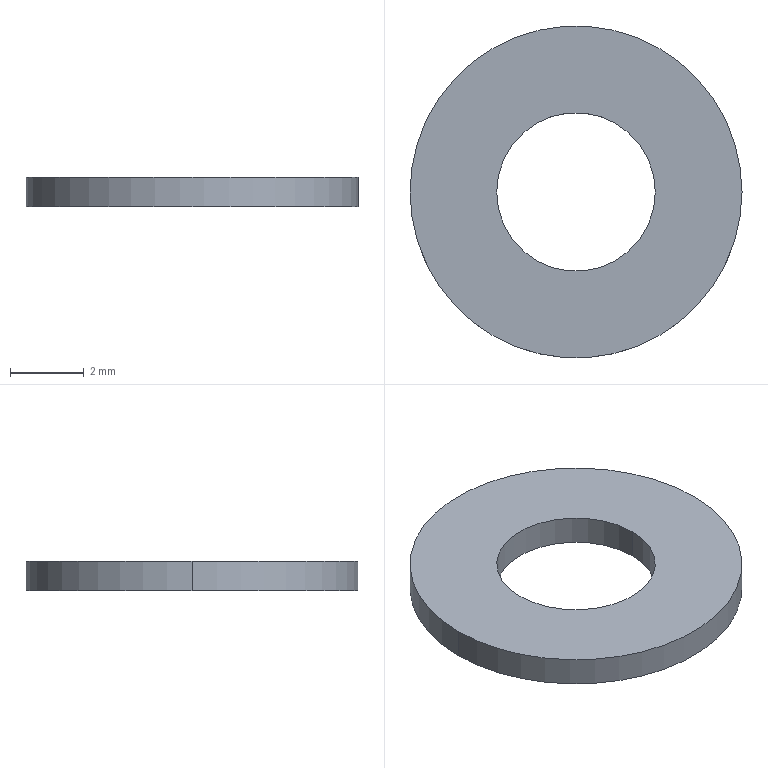Component | SolidWorks | FlatWasher4-1 | 1 solid | 6 faces | box 9 x 9 x 0.8 mm | volume 39 mm3 | cylinder 4 | plane 2 | commonest cylinder face diameters 4.3 x2 9 x2
build123d program:
from build123d import *

# Parameters (mm, degrees)
SKETCH1_R      = 4.5
SKETCH1_R_2    = 2.15
EXTRUDE1_DEPTH = 0.8


with BuildPart() as part:
    # Sketch1 → Extrude1 (new body)
    with BuildSketch(Plane.XY):
        Circle(SKETCH1_R)
        Circle(SKETCH1_R_2, mode=Mode.SUBTRACT)
    extrude(amount=EXTRUDE1_DEPTH)


solid = part.part

# Placed as in the assembly
solid = solid.moved(Location((-10, 5.5, 13.554), (0, 0, 0)))
STEP:
#1=CARTESIAN_POINT('',(-0.4783,0.2165,0.5651));
#2=VERTEX_POINT('',#1);
#3=CARTESIAN_POINT('',(-0.3091,0.2165,0.5651));
#4=VERTEX_POINT('',#3);
#5=CARTESIAN_POINT('',(-0.3937,0.2165,0.5651));
#6=DIRECTION('',(0.,0.,1.));
#7=DIRECTION('',(1.,0.,0.));
#8=AXIS2_PLACEMENT_3D('',#5,#6,#7);
#9=CIRCLE('',#8,0.08465);
#10=EDGE_CURVE('',#2,#4,#9,.T.);
#11=ORIENTED_EDGE('',*,*,#10,.T.);
#12=CARTESIAN_POINT('',(-0.3091,0.2165,0.5336));
#13=VERTEX_POINT('',#12);
#14=CARTESIAN_POINT('',(-0.3091,0.2165,0.5651));
#15=DIRECTION('',(0.,0.,-1.));
#16=VECTOR('',#15,39.37);
#17=LINE('',#14,#16);
#18=EDGE_CURVE('',#4,#13,#17,.T.);
#19=ORIENTED_EDGE('',*,*,#18,.T.);
#20=CARTESIAN_POINT('',(-0.4783,0.2165,0.5336));
#21=VERTEX_POINT('',#20);
#22=CARTESIAN_POINT('',(-0.3937,0.2165,0.5336));
#23=DIRECTION('',(0.,0.,1.));
#24=DIRECTION('',(1.,0.,0.));
#25=AXIS2_PLACEMENT_3D('',#22,#23,#24);
#26=CIRCLE('',#25,0.08465);
#27=EDGE_CURVE('',#21,#13,#26,.T.);
#28=ORIENTED_EDGE('',*,*,#27,.F.);
#29=CARTESIAN_POINT('',(-0.4783,0.2165,0.5651));
#30=DIRECTION('',(0.,0.,-1.));
#31=VECTOR('',#30,39.37);
#32=LINE('',#29,#31);
#33=EDGE_CURVE('',#2,#21,#32,.T.);
#34=ORIENTED_EDGE('',*,*,#33,.F.);
#35=EDGE_LOOP('',(#11,#19,#28,#34));
#36=FACE_OUTER_BOUND('',#35,.T.);
#37=CARTESIAN_POINT('',(-0.3937,0.2165,0.5651));
#38=DIRECTION('',(0.,0.,-1.));
#39=DIRECTION('',(-1.,0.,0.));
#40=AXIS2_PLACEMENT_3D('',#37,#38,#39);
#41=CYLINDRICAL_SURFACE('',#40,0.08465);
#42=ADVANCED_FACE('',(#36),#41,.F.);
#43=CARTESIAN_POINT('',(-0.2165,0.2165,0.5651));
#44=VERTEX_POINT('',#43);
#45=CARTESIAN_POINT('',(-0.5709,0.2165,0.5651));
#46=VERTEX_POINT('',#45);
#47=CARTESIAN_POINT('',(-0.3937,0.2165,0.5651));
#48=DIRECTION('',(0.,0.,1.));
#49=DIRECTION('',(1.,0.,0.));
#50=AXIS2_PLACEMENT_3D('',#47,#48,#49);
#51=CIRCLE('',#50,0.1772);
#52=EDGE_CURVE('',#44,#46,#51,.T.);
#53=ORIENTED_EDGE('',*,*,#52,.F.);
#54=CARTESIAN_POINT('',(-0.2165,0.2165,0.5336));
#55=VERTEX_POINT('',#54);
#56=CARTESIAN_POINT('',(-0.2165,0.2165,0.5651));
#57=DIRECTION('',(0.,0.,-1.));
#58=VECTOR('',#57,39.37);
#59=LINE('',#56,#58);
#60=EDGE_CURVE('',#44,#55,#59,.T.);
#61=ORIENTED_EDGE('',*,*,#60,.T.);
#62=CARTESIAN_POINT('',(-0.5709,0.2165,0.5336));
#63=VERTEX_POINT('',#62);
#64=CARTESIAN_POINT('',(-0.3937,0.2165,0.5336));
#65=DIRECTION('',(0.,0.,1.));
#66=DIRECTION('',(1.,0.,0.));
#67=AXIS2_PLACEMENT_3D('',#64,#65,#66);
#68=CIRCLE('',#67,0.1772);
#69=EDGE_CURVE('',#55,#63,#68,.T.);
#70=ORIENTED_EDGE('',*,*,#69,.T.);
#71=CARTESIAN_POINT('',(-0.5709,0.2165,0.5651));
#72=DIRECTION('',(0.,0.,-1.));
#73=VECTOR('',#72,39.37);
#74=LINE('',#71,#73);
#75=EDGE_CURVE('',#46,#63,#74,.T.);
#76=ORIENTED_EDGE('',*,*,#75,.F.);
#77=EDGE_LOOP('',(#53,#61,#70,#76));
#78=FACE_OUTER_BOUND('',#77,.T.);
#79=CARTESIAN_POINT('',(-0.3937,0.2165,0.5651));
#80=DIRECTION('',(0.,0.,-1.));
#81=DIRECTION('',(-1.,0.,0.));
#82=AXIS2_PLACEMENT_3D('',#79,#80,#81);
#83=CYLINDRICAL_SURFACE('',#82,0.1772);
#84=ADVANCED_FACE('',(#78),#83,.T.);
#85=CARTESIAN_POINT('',(-0.3937,0.2165,0.5651));
#86=DIRECTION('',(0.,0.,1.));
#87=DIRECTION('',(1.,0.,0.));
#88=AXIS2_PLACEMENT_3D('',#85,#86,#87);
#89=CIRCLE('',#88,0.1772);
#90=EDGE_CURVE('',#46,#44,#89,.T.);
#91=ORIENTED_EDGE('',*,*,#90,.T.);
#92=ORIENTED_EDGE('',*,*,#52,.T.);
#93=EDGE_LOOP('',(#91,#92));
#94=FACE_OUTER_BOUND('',#93,.T.);
#95=ORIENTED_EDGE('',*,*,#10,.F.);
#96=CARTESIAN_POINT('',(-0.3937,0.2165,0.5651));
#97=DIRECTION('',(0.,0.,1.));
#98=DIRECTION('',(1.,0.,0.));
#99=AXIS2_PLACEMENT_3D('',#96,#97,#98);
#100=CIRCLE('',#99,0.08465);
#101=EDGE_CURVE('',#4,#2,#100,.T.);
#102=ORIENTED_EDGE('',*,*,#101,.F.);
#103=EDGE_LOOP('',(#95,#102));
#104=FACE_BOUND('',#103,.T.);
#105=CARTESIAN_POINT('',(-0.3937,0.2165,0.5651));
#106=DIRECTION('',(0.,0.,1.));
#107=DIRECTION('',(1.,0.,0.));
#108=AXIS2_PLACEMENT_3D('',#105,#106,#107);
#109=PLANE('',#108);
#110=ADVANCED_FACE('',(#94,#104),#109,.T.);
#111=CARTESIAN_POINT('',(-0.3937,0.2165,0.5336));
#112=DIRECTION('',(0.,0.,1.));
#113=DIRECTION('',(1.,0.,0.));
#114=AXIS2_PLACEMENT_3D('',#111,#112,#113);
#115=CIRCLE('',#114,0.1772);
#116=EDGE_CURVE('',#63,#55,#115,.T.);
#117=ORIENTED_EDGE('',*,*,#116,.F.);
#118=ORIENTED_EDGE('',*,*,#69,.F.);
#119=EDGE_LOOP('',(#117,#118));
#120=FACE_OUTER_BOUND('',#119,.T.);
#121=ORIENTED_EDGE('',*,*,#27,.T.);
#122=CARTESIAN_POINT('',(-0.3937,0.2165,0.5336));
#123=DIRECTION('',(0.,0.,1.));
#124=DIRECTION('',(1.,0.,0.));
#125=AXIS2_PLACEMENT_3D('',#122,#123,#124);
#126=CIRCLE('',#125,0.08465);
#127=EDGE_CURVE('',#13,#21,#126,.T.);
#128=ORIENTED_EDGE('',*,*,#127,.T.);
#129=EDGE_LOOP('',(#121,#128));
#130=FACE_BOUND('',#129,.T.);
#131=CARTESIAN_POINT('',(-0.3937,0.2165,0.5336));
#132=DIRECTION('',(0.,0.,1.));
#133=DIRECTION('',(1.,0.,0.));
#134=AXIS2_PLACEMENT_3D('',#131,#132,#133);
#135=PLANE('',#134);
#136=ADVANCED_FACE('',(#120,#130),#135,.F.);
#137=ORIENTED_EDGE('',*,*,#60,.F.);
#138=ORIENTED_EDGE('',*,*,#90,.F.);
#139=ORIENTED_EDGE('',*,*,#75,.T.);
#140=ORIENTED_EDGE('',*,*,#116,.T.);
#141=EDGE_LOOP('',(#137,#138,#139,#140));
#142=FACE_OUTER_BOUND('',#141,.T.);
#143=CARTESIAN_POINT('',(-0.3937,0.2165,0.5651));
#144=DIRECTION('',(0.,0.,-1.));
#145=DIRECTION('',(-1.,0.,0.));
#146=AXIS2_PLACEMENT_3D('',#143,#144,#145);
#147=CYLINDRICAL_SURFACE('',#146,0.1772);
#148=ADVANCED_FACE('',(#142),#147,.T.);
#149=ORIENTED_EDGE('',*,*,#18,.F.);
#150=ORIENTED_EDGE('',*,*,#101,.T.);
#151=ORIENTED_EDGE('',*,*,#33,.T.);
#152=ORIENTED_EDGE('',*,*,#127,.F.);
#153=EDGE_LOOP('',(#149,#150,#151,#152));
#154=FACE_OUTER_BOUND('',#153,.T.);
#155=CARTESIAN_POINT('',(-0.3937,0.2165,0.5651));
#156=DIRECTION('',(0.,0.,-1.));
#157=DIRECTION('',(-1.,0.,0.));
#158=AXIS2_PLACEMENT_3D('',#155,#156,#157);
#159=CYLINDRICAL_SURFACE('',#158,0.08465);
#160=ADVANCED_FACE('',(#154),#159,.F.);
#161=CLOSED_SHELL('',(#42,#84,#110,#136,#148,#160));
#162=MANIFOLD_SOLID_BREP('',#161);
#163=CARTESIAN_POINT('',(0.,0.,0.));
#164=DIRECTION('',(0.,0.,1.));
#165=DIRECTION('',(1.,0.,0.));
#166=AXIS2_PLACEMENT_3D('',#163,#164,#165);
#167=(LENGTH_UNIT()NAMED_UNIT(*)SI_UNIT($,.METRE.));
#168=LENGTH_MEASURE_WITH_UNIT(LENGTH_MEASURE(0.0254),#167);
#169=DIMENSIONAL_EXPONENTS(1.,0.,0.,0.,0.,0.,0.);
#170=(CONVERSION_BASED_UNIT('',#168)LENGTH_UNIT()NAMED_UNIT(#169));
#171=UNCERTAINTY_MEASURE_WITH_UNIT(LENGTH_MEASURE(0.00001),#170,'','');
#172=(NAMED_UNIT(*)PLANE_ANGLE_UNIT()SI_UNIT($,.RADIAN.));
#173=(NAMED_UNIT(*)SI_UNIT($,.STERADIAN.)SOLID_ANGLE_UNIT());
#174=(GEOMETRIC_REPRESENTATION_CONTEXT(3)GLOBAL_UNCERTAINTY_ASSIGNED_CONTEXT((#171))GLOBAL_UNIT_ASSIGNED_CONTEXT((#170,#172,#173))REPRESENTATION_CONTEXT('',''));
#175=ADVANCED_BREP_SHAPE_REPRESENTATION('',(#162,#166),#174);
#176=COLOUR_RGB('',0.7922,0.8196,0.9333);
#177=FILL_AREA_STYLE_COLOUR('',#176);
#178=FILL_AREA_STYLE('',(#177));
#179=SURFACE_STYLE_FILL_AREA(#178);
#180=SURFACE_SIDE_STYLE('',(#179));
#181=SURFACE_STYLE_USAGE(.BOTH.,#180);
#182=PRESENTATION_STYLE_ASSIGNMENT((#181));
#183=STYLED_ITEM('',(#182),#162);
#184=PRESENTATION_LAYER_ASSIGNMENT('','',(#183));
#185=(LENGTH_UNIT()NAMED_UNIT(*)SI_UNIT($,.METRE.));
#186=LENGTH_MEASURE_WITH_UNIT(LENGTH_MEASURE(0.0254),#185);
#187=DIMENSIONAL_EXPONENTS(1.,0.,0.,0.,0.,0.,0.);
#188=(CONVERSION_BASED_UNIT('',#186)LENGTH_UNIT()NAMED_UNIT(#187));
#189=UNCERTAINTY_MEASURE_WITH_UNIT(LENGTH_MEASURE(0.00001),#188,'','');
#190=(NAMED_UNIT(*)PLANE_ANGLE_UNIT()SI_UNIT($,.RADIAN.));
#191=(NAMED_UNIT(*)SI_UNIT($,.STERADIAN.)SOLID_ANGLE_UNIT());
#192=(GEOMETRIC_REPRESENTATION_CONTEXT(3)GLOBAL_UNCERTAINTY_ASSIGNED_CONTEXT((#189))GLOBAL_UNIT_ASSIGNED_CONTEXT((#188,#190,#191))REPRESENTATION_CONTEXT('',''));
#193=MECHANICAL_DESIGN_GEOMETRIC_PRESENTATION_REPRESENTATION('',(#183),#192);